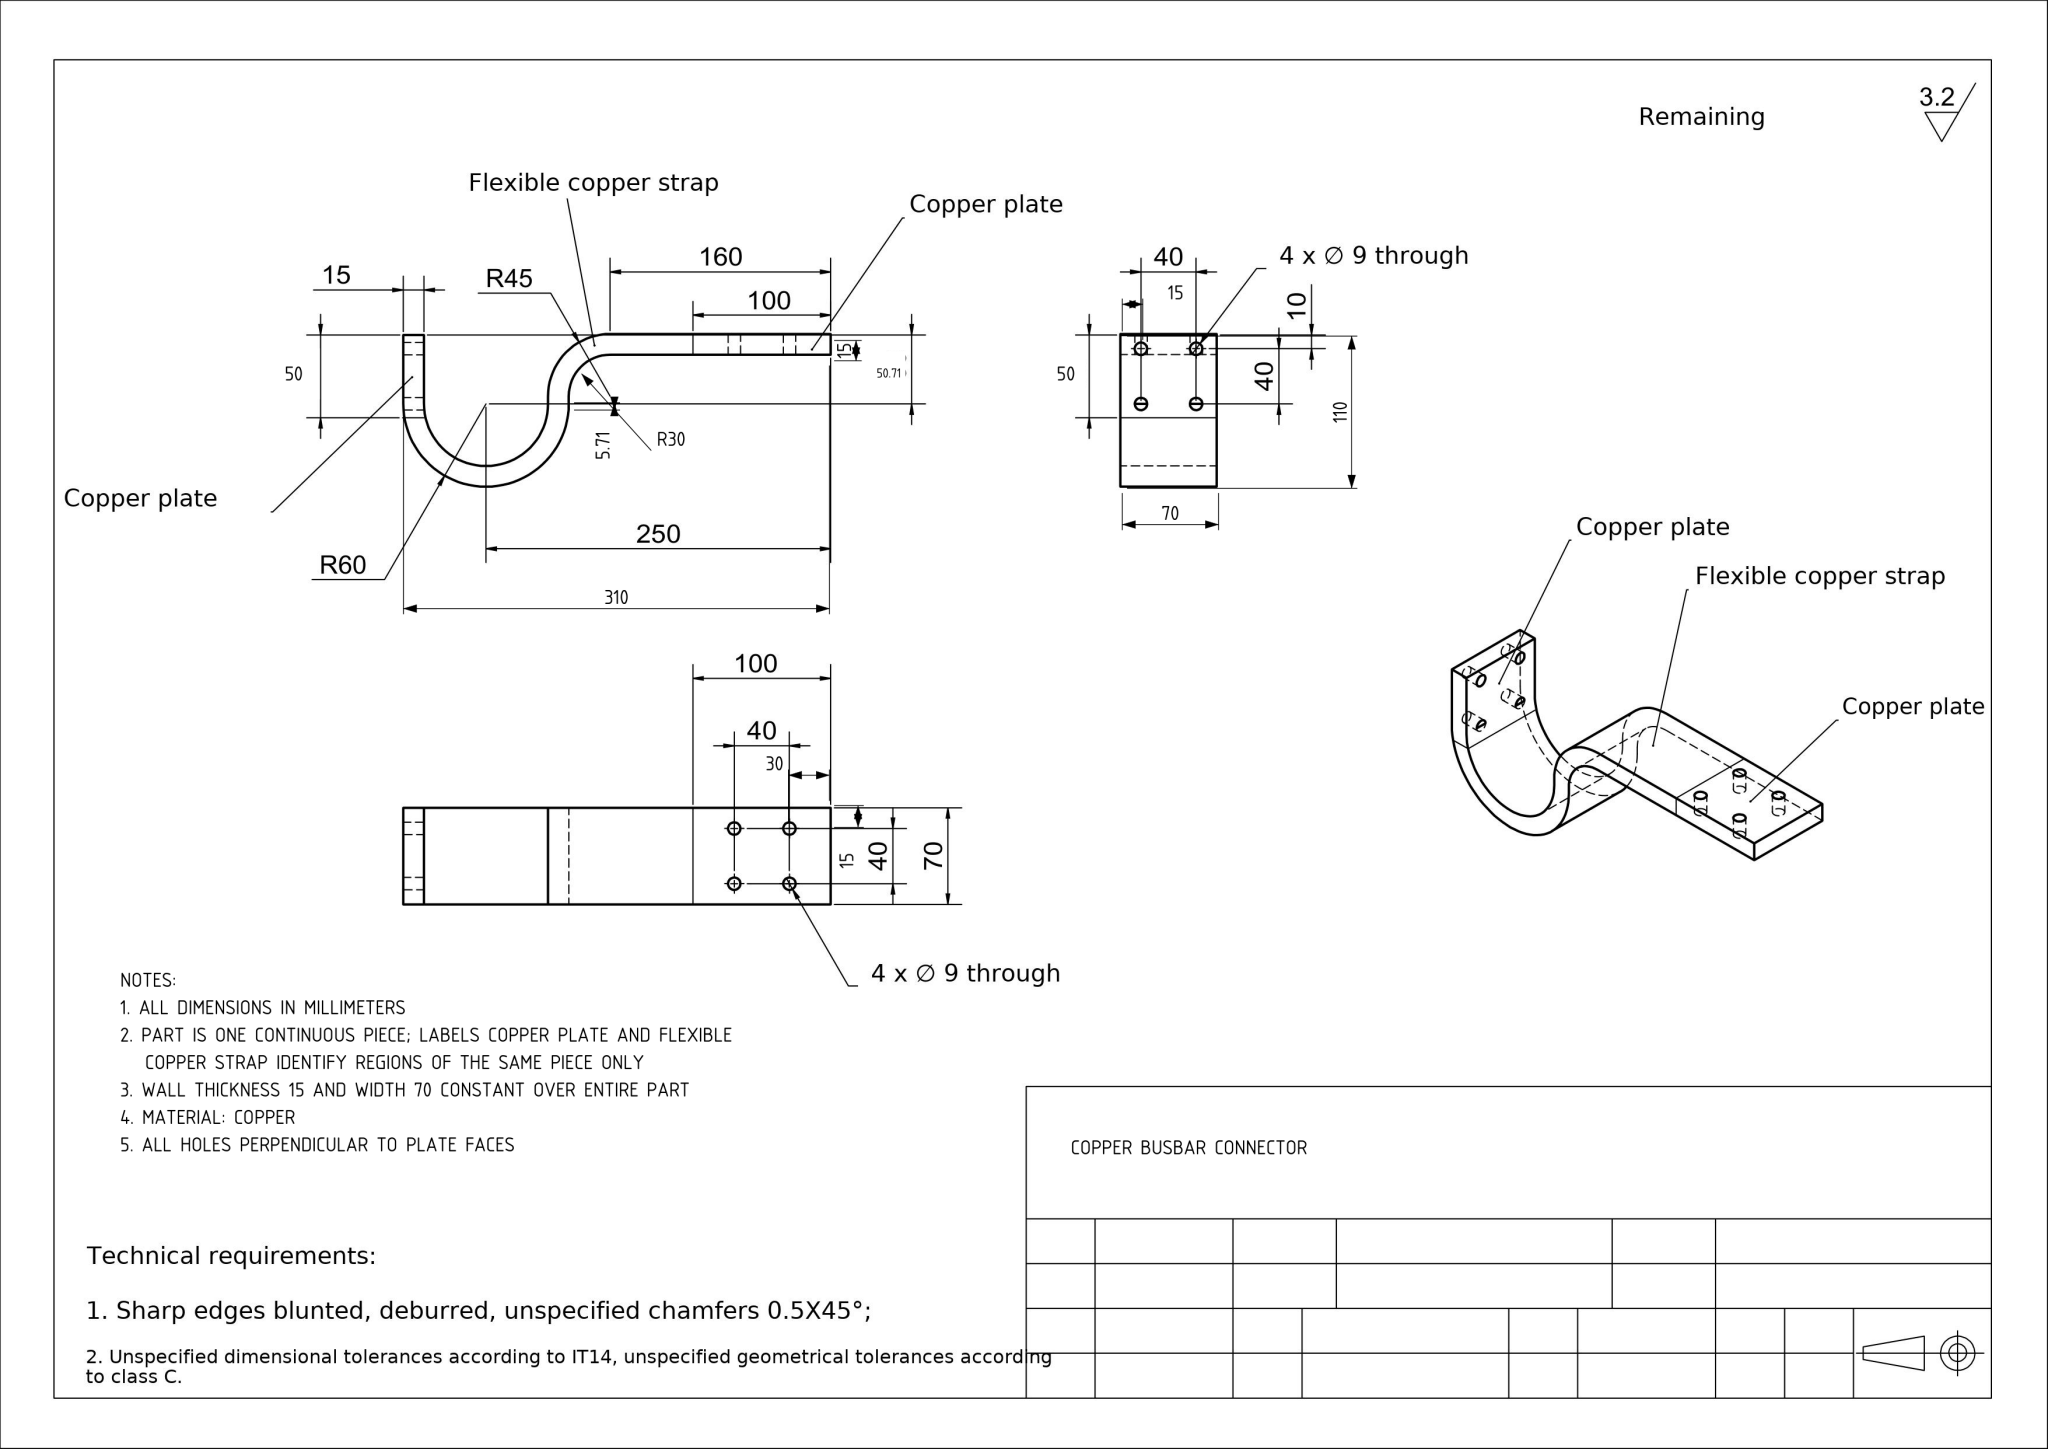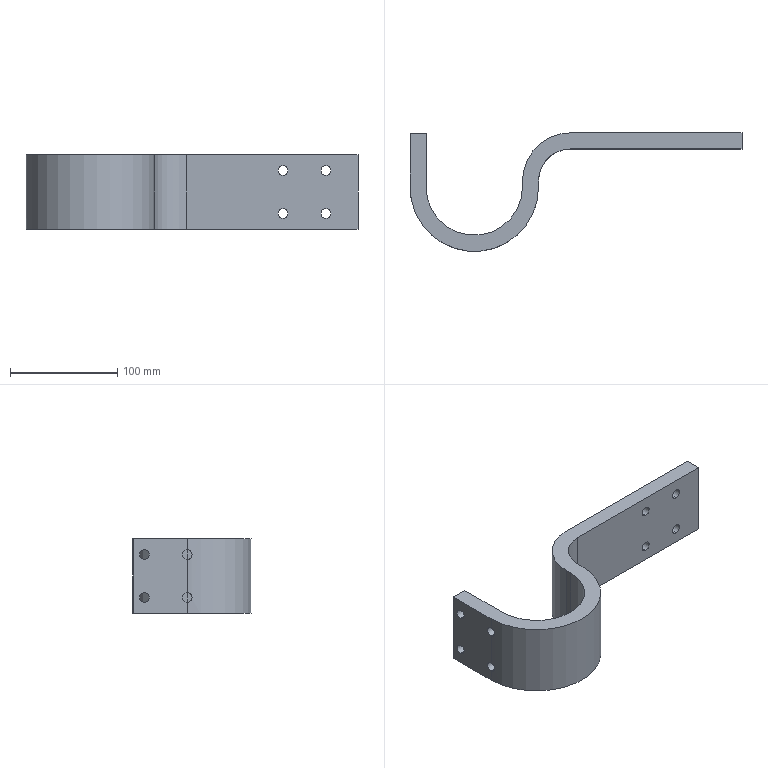Part | NX | mm | 1 solid | 32 faces | box 310 x 110.71 x 70 mm | volume 453900 mm3 | cylinder 20 | plane 12 | commonest cylinder face diameters 9 x16 90 x2 120 x1 60 x1